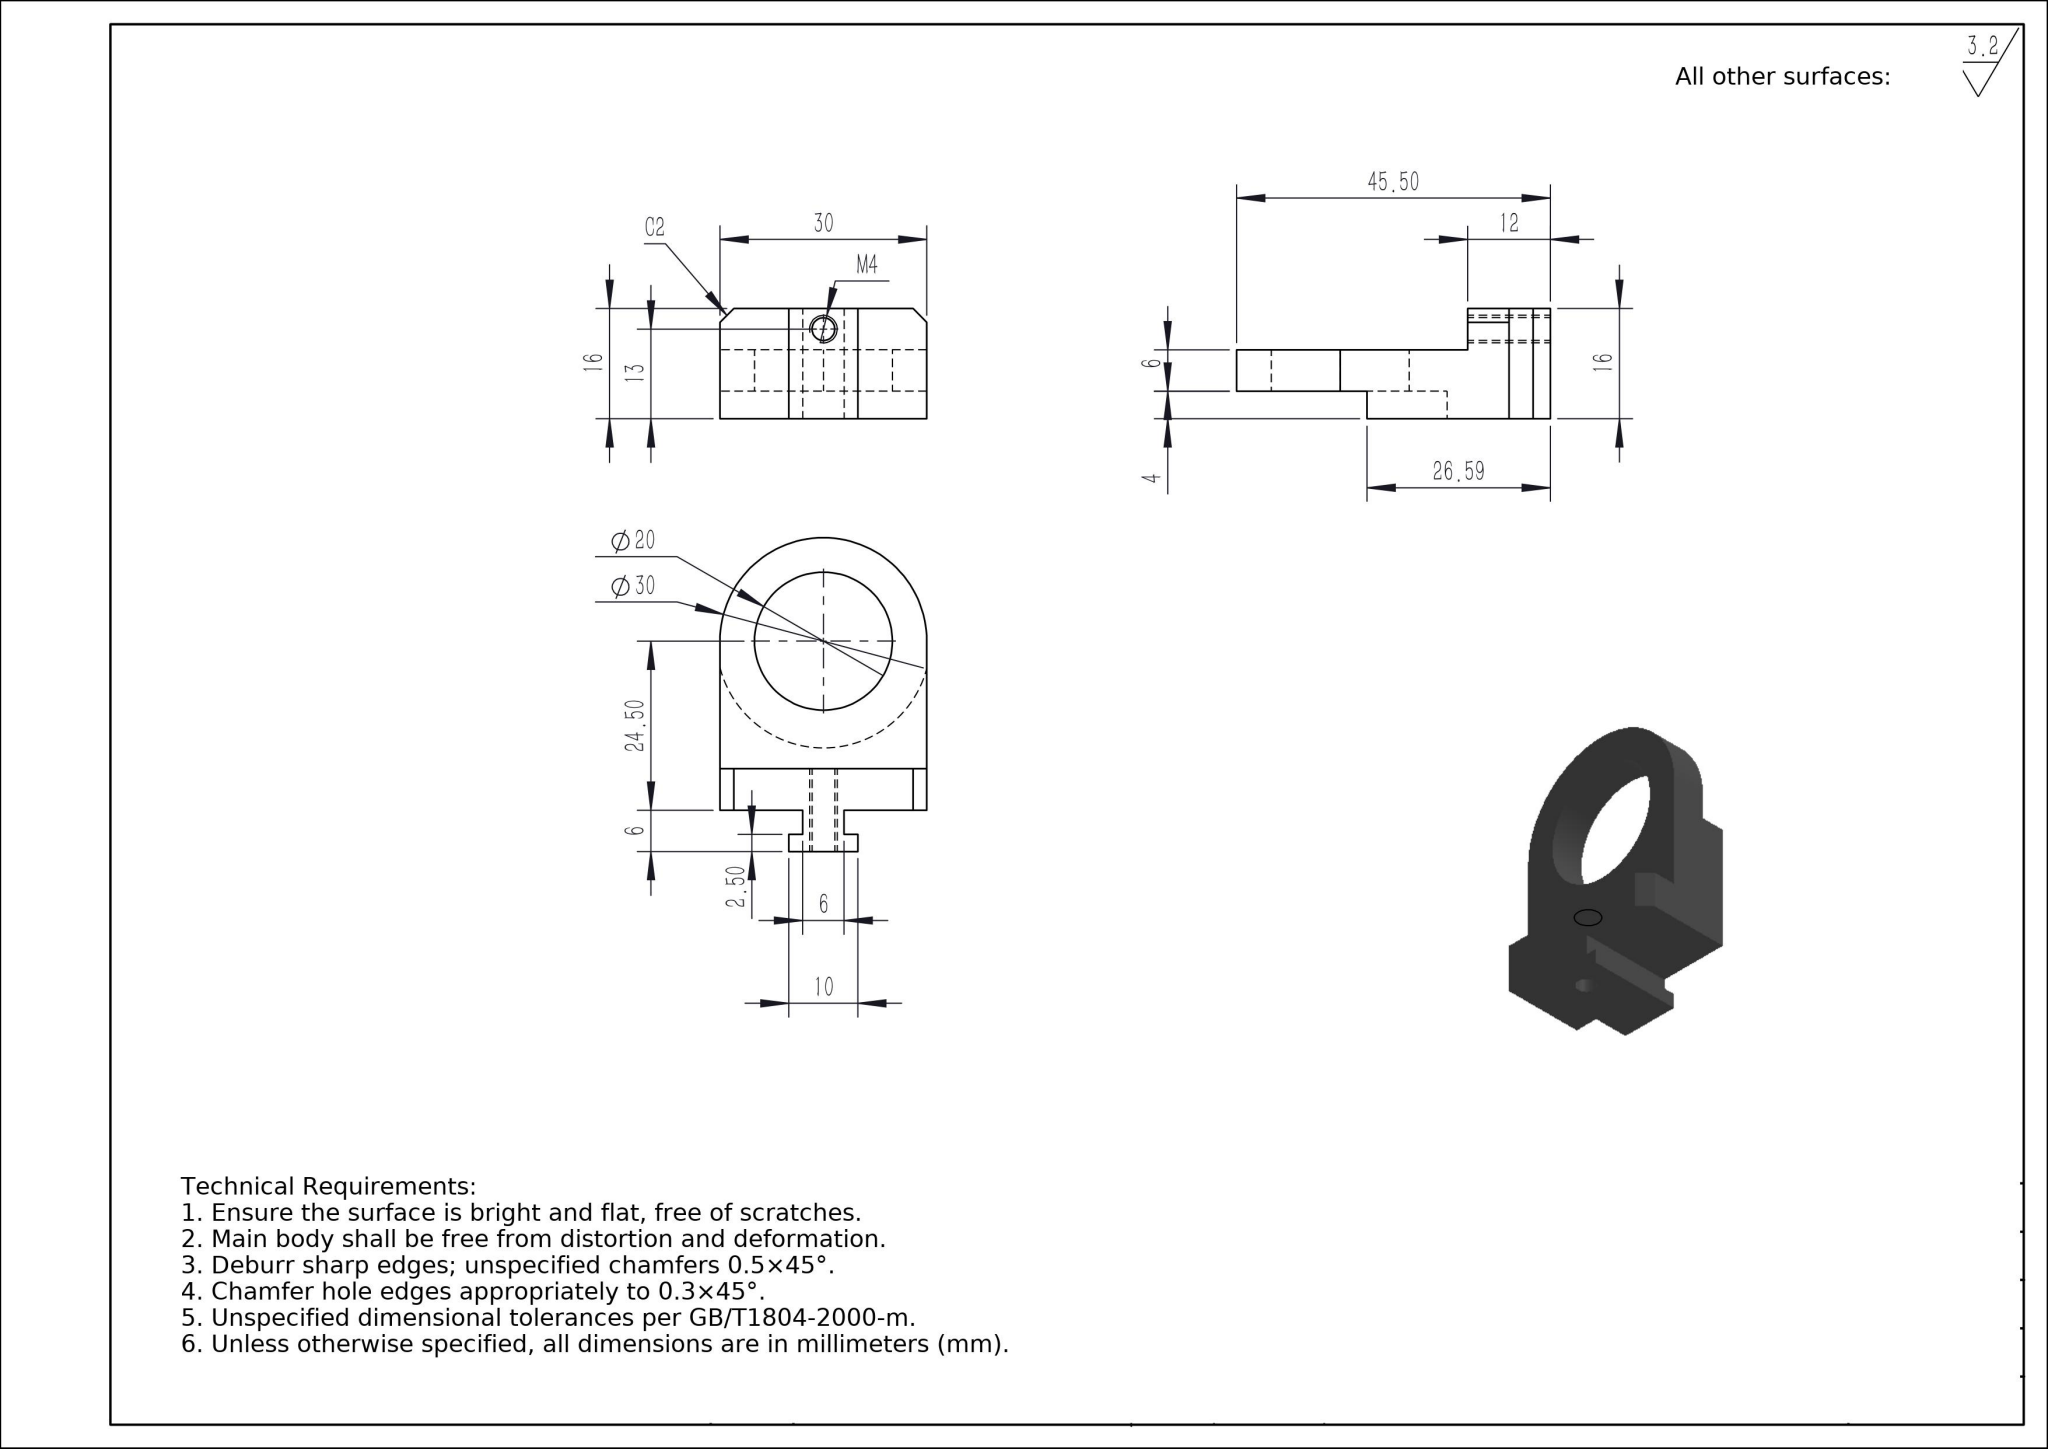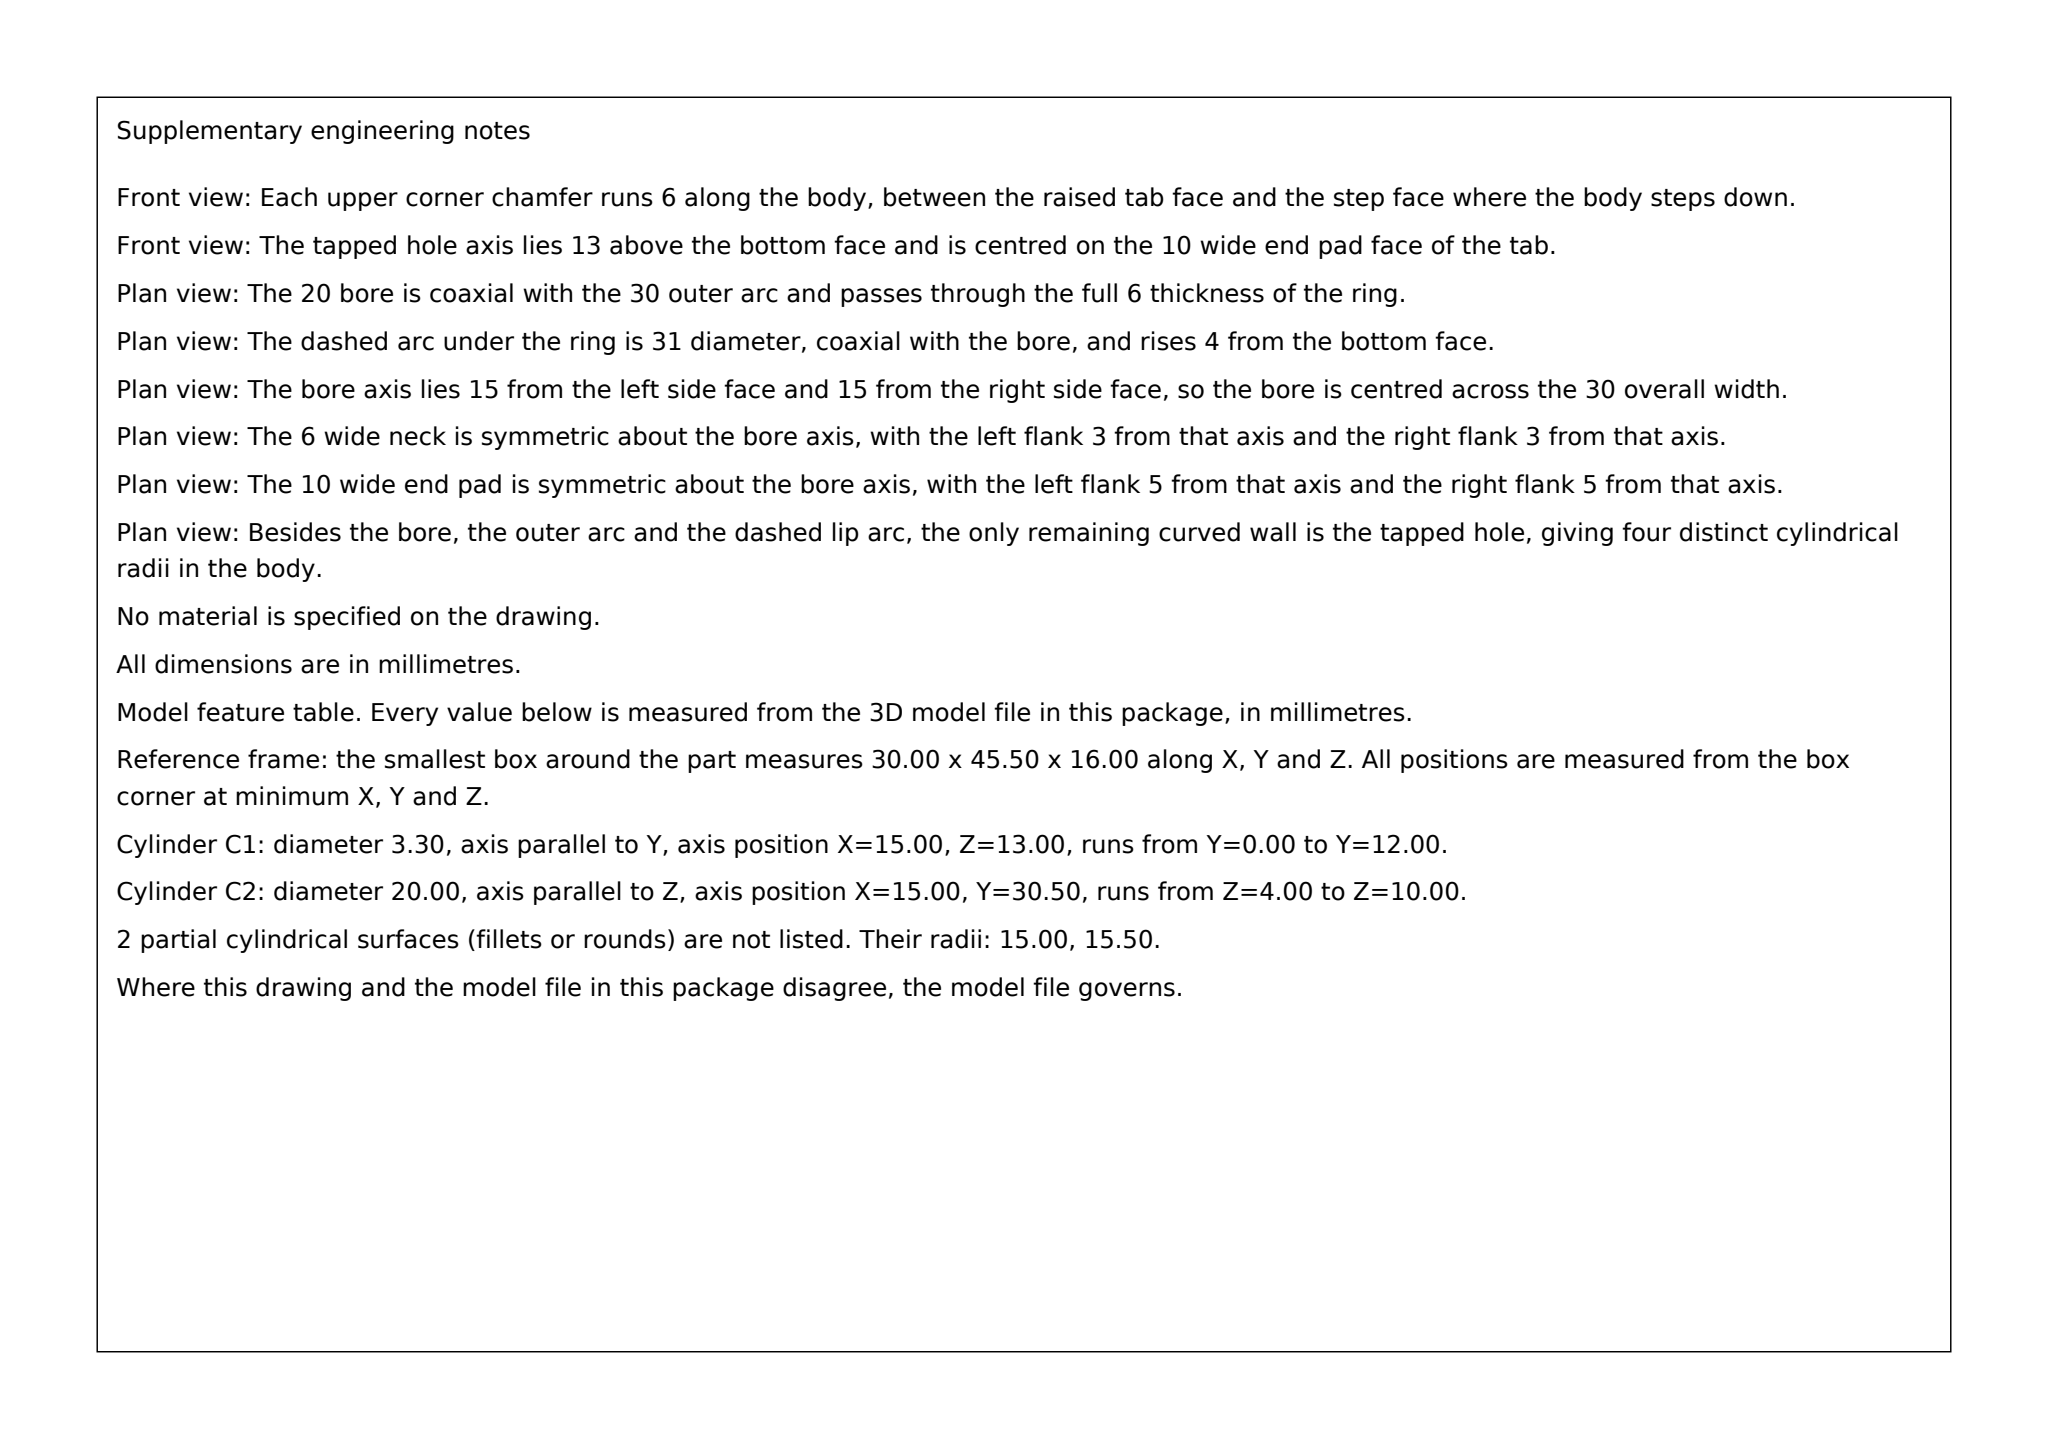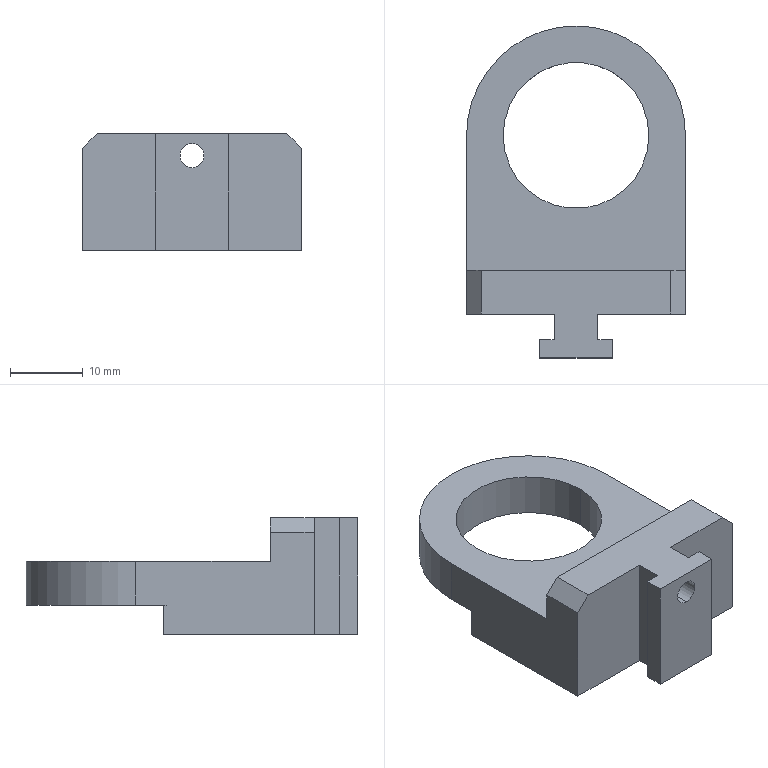Part | SolidWorks | mm | 1 solid | 25 faces | box 30 x 45.5 x 16 mm | volume 7776 mm3 | plane 18 | cylinder 7 | commonest cylinder face diameters 3.3 x2 20 x2 30 x2 31 x1
Drawing notes:
M4 TAPPED HOLE: 15 FROM EACH END OF 30 WIDTH (ON CL), 13 UP | from the solid: cylinder dia 3.3 axis y at x=15.0, z=13.0; bbox x=30.0 so x=15 is mid-width
R15.50 CONCAVE ARC COAXIAL W/ Ø30 BOSS, 4 DEEP FROM BOTTOM FACE | from the solid: concave arc dia 31.0 (R15.50), axis z at (15.0,30.5), from z=0.0 to z=4.0, 151 deg, same center as Ø30 convex arc and Ø20 bore
STEP:
#1=CARTESIAN_POINT('',(0.,-25.75,11.35));
#2=VERTEX_POINT('',#1);
#3=CARTESIAN_POINT('',(0.,-25.75,14.65));
#4=VERTEX_POINT('',#3);
#5=CARTESIAN_POINT('',(0.,-25.75,13.));
#6=DIRECTION('',(0.,1.,0.));
#7=DIRECTION('',(0.,0.,1.));
#8=AXIS2_PLACEMENT_3D('',#5,#6,#7);
#9=CIRCLE('',#8,1.65);
#10=EDGE_CURVE('',#2,#4,#9,.T.);
#11=ORIENTED_EDGE('',*,*,#10,.F.);
#12=CARTESIAN_POINT('',(0.,-13.75,11.35));
#13=VERTEX_POINT('',#12);
#14=CARTESIAN_POINT('',(0.,-13.75,11.35));
#15=DIRECTION('',(0.,1.,0.));
#16=VECTOR('',#15,1000.);
#17=LINE('',#14,#16);
#18=EDGE_CURVE('',#2,#13,#17,.T.);
#19=ORIENTED_EDGE('',*,*,#18,.T.);
#20=CARTESIAN_POINT('',(0.,-13.75,14.65));
#21=VERTEX_POINT('',#20);
#22=CARTESIAN_POINT('',(0.,-13.75,13.));
#23=DIRECTION('',(0.,1.,0.));
#24=DIRECTION('',(0.,0.,1.));
#25=AXIS2_PLACEMENT_3D('',#22,#23,#24);
#26=CIRCLE('',#25,1.65);
#27=EDGE_CURVE('',#13,#21,#26,.T.);
#28=ORIENTED_EDGE('',*,*,#27,.T.);
#29=CARTESIAN_POINT('',(0.,-13.75,14.65));
#30=DIRECTION('',(0.,1.,0.));
#31=VECTOR('',#30,1000.);
#32=LINE('',#29,#31);
#33=EDGE_CURVE('',#4,#21,#32,.T.);
#34=ORIENTED_EDGE('',*,*,#33,.F.);
#35=EDGE_LOOP('',(#11,#19,#28,#34));
#36=FACE_OUTER_BOUND('',#35,.T.);
#37=CARTESIAN_POINT('',(0.,-13.75,13.));
#38=DIRECTION('',(0.,1.,0.));
#39=DIRECTION('',(0.,0.,1.));
#40=AXIS2_PLACEMENT_3D('',#37,#38,#39);
#41=CYLINDRICAL_SURFACE('',#40,1.65);
#42=ADVANCED_FACE('',(#36),#41,.F.);
#43=CARTESIAN_POINT('',(-10.,4.75,4.));
#44=VERTEX_POINT('',#43);
#45=CARTESIAN_POINT('',(10.,4.75,4.));
#46=VERTEX_POINT('',#45);
#47=CARTESIAN_POINT('',(0.,4.75,4.));
#48=DIRECTION('',(0.,0.,1.));
#49=DIRECTION('',(-1.,0.,0.));
#50=AXIS2_PLACEMENT_3D('',#47,#48,#49);
#51=CIRCLE('',#50,10.);
#52=EDGE_CURVE('',#44,#46,#51,.T.);
#53=ORIENTED_EDGE('',*,*,#52,.F.);
#54=CARTESIAN_POINT('',(-10.,4.75,10.));
#55=VERTEX_POINT('',#54);
#56=CARTESIAN_POINT('',(-10.,4.75,-5.));
#57=DIRECTION('',(0.,0.,1.));
#58=VECTOR('',#57,1000.);
#59=LINE('',#56,#58);
#60=EDGE_CURVE('',#44,#55,#59,.T.);
#61=ORIENTED_EDGE('',*,*,#60,.T.);
#62=CARTESIAN_POINT('',(10.,4.75,10.));
#63=VERTEX_POINT('',#62);
#64=CARTESIAN_POINT('',(0.,4.75,10.));
#65=DIRECTION('',(0.,0.,1.));
#66=DIRECTION('',(1.,0.,0.));
#67=AXIS2_PLACEMENT_3D('',#64,#65,#66);
#68=CIRCLE('',#67,10.);
#69=EDGE_CURVE('',#55,#63,#68,.T.);
#70=ORIENTED_EDGE('',*,*,#69,.T.);
#71=CARTESIAN_POINT('',(10.,4.75,-5.));
#72=DIRECTION('',(0.,0.,1.));
#73=VECTOR('',#72,1000.);
#74=LINE('',#71,#73);
#75=EDGE_CURVE('',#46,#63,#74,.T.);
#76=ORIENTED_EDGE('',*,*,#75,.F.);
#77=EDGE_LOOP('',(#53,#61,#70,#76));
#78=FACE_OUTER_BOUND('',#77,.T.);
#79=CARTESIAN_POINT('',(0.,4.75,-5.));
#80=DIRECTION('',(0.,0.,1.));
#81=DIRECTION('',(1.,0.,0.));
#82=AXIS2_PLACEMENT_3D('',#79,#80,#81);
#83=CYLINDRICAL_SURFACE('',#82,10.);
#84=ADVANCED_FACE('',(#78),#83,.F.);
#85=CARTESIAN_POINT('',(-3.,-19.75,16.));
#86=VERTEX_POINT('',#85);
#87=CARTESIAN_POINT('',(-3.,-19.75,0.));
#88=VERTEX_POINT('',#87);
#89=CARTESIAN_POINT('',(-3.,-19.75,-0.));
#90=DIRECTION('',(0.,0.,-1.));
#91=VECTOR('',#90,1000.);
#92=LINE('',#89,#91);
#93=EDGE_CURVE('',#86,#88,#92,.T.);
#94=ORIENTED_EDGE('',*,*,#93,.F.);
#95=CARTESIAN_POINT('',(-13.,-19.75,16.));
#96=VERTEX_POINT('',#95);
#97=CARTESIAN_POINT('',(-15.,-19.75,16.));
#98=DIRECTION('',(1.,0.,0.));
#99=VECTOR('',#98,1000.);
#100=LINE('',#97,#99);
#101=EDGE_CURVE('',#96,#86,#100,.T.);
#102=ORIENTED_EDGE('',*,*,#101,.F.);
#103=CARTESIAN_POINT('',(-15.,-19.75,14.));
#104=VERTEX_POINT('',#103);
#105=CARTESIAN_POINT('',(-13.,-19.75,16.));
#106=DIRECTION('',(-0.7071,-0.,-0.7071));
#107=VECTOR('',#106,1000.);
#108=LINE('',#105,#107);
#109=EDGE_CURVE('',#96,#104,#108,.T.);
#110=ORIENTED_EDGE('',*,*,#109,.T.);
#111=CARTESIAN_POINT('',(-15.,-19.75,0.));
#112=VERTEX_POINT('',#111);
#113=CARTESIAN_POINT('',(-15.,-19.75,10.));
#114=DIRECTION('',(0.,0.,-1.));
#115=VECTOR('',#114,1000.);
#116=LINE('',#113,#115);
#117=EDGE_CURVE('',#104,#112,#116,.T.);
#118=ORIENTED_EDGE('',*,*,#117,.T.);
#119=CARTESIAN_POINT('',(15.,-19.75,0.));
#120=DIRECTION('',(1.,0.,0.));
#121=VECTOR('',#120,1000.);
#122=LINE('',#119,#121);
#123=EDGE_CURVE('',#112,#88,#122,.T.);
#124=ORIENTED_EDGE('',*,*,#123,.T.);
#125=EDGE_LOOP('',(#94,#102,#110,#118,#124));
#126=FACE_OUTER_BOUND('',#125,.T.);
#127=CARTESIAN_POINT('',(15.,-19.75,10.));
#128=DIRECTION('',(-0.,1.,0.));
#129=DIRECTION('',(-1.,-0.,0.));
#130=AXIS2_PLACEMENT_3D('',#127,#128,#129);
#131=PLANE('',#130);
#132=ADVANCED_FACE('',(#126),#131,.F.);
#133=CARTESIAN_POINT('',(3.,-19.75,0.));
#134=VERTEX_POINT('',#133);
#135=CARTESIAN_POINT('',(3.,-19.75,16.));
#136=VERTEX_POINT('',#135);
#137=CARTESIAN_POINT('',(3.,-19.75,-0.));
#138=DIRECTION('',(0.,0.,1.));
#139=VECTOR('',#138,1000.);
#140=LINE('',#137,#139);
#141=EDGE_CURVE('',#134,#136,#140,.T.);
#142=ORIENTED_EDGE('',*,*,#141,.F.);
#143=CARTESIAN_POINT('',(15.,-19.75,0.));
#144=VERTEX_POINT('',#143);
#145=CARTESIAN_POINT('',(15.,-19.75,0.));
#146=DIRECTION('',(1.,0.,0.));
#147=VECTOR('',#146,1000.);
#148=LINE('',#145,#147);
#149=EDGE_CURVE('',#134,#144,#148,.T.);
#150=ORIENTED_EDGE('',*,*,#149,.T.);
#151=CARTESIAN_POINT('',(15.,-19.75,14.));
#152=VERTEX_POINT('',#151);
#153=CARTESIAN_POINT('',(15.,-19.75,10.));
#154=DIRECTION('',(0.,0.,-1.));
#155=VECTOR('',#154,1000.);
#156=LINE('',#153,#155);
#157=EDGE_CURVE('',#152,#144,#156,.T.);
#158=ORIENTED_EDGE('',*,*,#157,.F.);
#159=CARTESIAN_POINT('',(13.,-19.75,16.));
#160=VERTEX_POINT('',#159);
#161=CARTESIAN_POINT('',(13.,-19.75,16.));
#162=DIRECTION('',(-0.7071,-0.,0.7071));
#163=VECTOR('',#162,1000.);
#164=LINE('',#161,#163);
#165=EDGE_CURVE('',#152,#160,#164,.T.);
#166=ORIENTED_EDGE('',*,*,#165,.T.);
#167=CARTESIAN_POINT('',(-15.,-19.75,16.));
#168=DIRECTION('',(1.,0.,0.));
#169=VECTOR('',#168,1000.);
#170=LINE('',#167,#169);
#171=EDGE_CURVE('',#136,#160,#170,.T.);
#172=ORIENTED_EDGE('',*,*,#171,.F.);
#173=EDGE_LOOP('',(#142,#150,#158,#166,#172));
#174=FACE_OUTER_BOUND('',#173,.T.);
#175=CARTESIAN_POINT('',(15.,-19.75,10.));
#176=DIRECTION('',(-0.,1.,0.));
#177=DIRECTION('',(-1.,-0.,0.));
#178=AXIS2_PLACEMENT_3D('',#175,#176,#177);
#179=PLANE('',#178);
#180=ADVANCED_FACE('',(#174),#179,.F.);
#181=CARTESIAN_POINT('',(-0.,19.75,4.));
#182=VERTEX_POINT('',#181);
#183=CARTESIAN_POINT('',(-0.,19.75,10.));
#184=VERTEX_POINT('',#183);
#185=CARTESIAN_POINT('',(-0.,19.75,10.));
#186=DIRECTION('',(0.,0.,1.));
#187=VECTOR('',#186,1000.);
#188=LINE('',#185,#187);
#189=EDGE_CURVE('',#182,#184,#188,.T.);
#190=ORIENTED_EDGE('',*,*,#189,.F.);
#191=CARTESIAN_POINT('',(-15.,4.75,4.));
#192=VERTEX_POINT('',#191);
#193=CARTESIAN_POINT('',(0.,4.75,4.));
#194=DIRECTION('',(0.,0.,1.));
#195=DIRECTION('',(-1.,-0.,0.));
#196=AXIS2_PLACEMENT_3D('',#193,#194,#195);
#197=CIRCLE('',#196,15.);
#198=EDGE_CURVE('',#182,#192,#197,.T.);
#199=ORIENTED_EDGE('',*,*,#198,.T.);
#200=CARTESIAN_POINT('',(-15.,4.75,10.));
#201=VERTEX_POINT('',#200);
#202=CARTESIAN_POINT('',(-15.,4.75,10.));
#203=DIRECTION('',(0.,0.,-1.));
#204=VECTOR('',#203,1000.);
#205=LINE('',#202,#204);
#206=EDGE_CURVE('',#201,#192,#205,.T.);
#207=ORIENTED_EDGE('',*,*,#206,.F.);
#208=CARTESIAN_POINT('',(0.,4.75,10.));
#209=DIRECTION('',(0.,0.,1.));
#210=DIRECTION('',(1.,0.,0.));
#211=AXIS2_PLACEMENT_3D('',#208,#209,#210);
#212=CIRCLE('',#211,15.);
#213=EDGE_CURVE('',#184,#201,#212,.T.);
#214=ORIENTED_EDGE('',*,*,#213,.F.);
#215=EDGE_LOOP('',(#190,#199,#207,#214));
#216=FACE_OUTER_BOUND('',#215,.T.);
#217=CARTESIAN_POINT('',(0.,4.75,10.));
#218=DIRECTION('',(0.,0.,-1.));
#219=DIRECTION('',(-1.,0.,0.));
#220=AXIS2_PLACEMENT_3D('',#217,#218,#219);
#221=CYLINDRICAL_SURFACE('',#220,15.);
#222=ADVANCED_FACE('',(#216),#221,.T.);
#223=CARTESIAN_POINT('',(15.,4.75,4.));
#224=VERTEX_POINT('',#223);
#225=CARTESIAN_POINT('',(15.,4.75,10.));
#226=VERTEX_POINT('',#225);
#227=CARTESIAN_POINT('',(15.,4.75,10.));
#228=DIRECTION('',(0.,0.,1.));
#229=VECTOR('',#228,1000.);
#230=LINE('',#227,#229);
#231=EDGE_CURVE('',#224,#226,#230,.T.);
#232=ORIENTED_EDGE('',*,*,#231,.F.);
#233=CARTESIAN_POINT('',(0.,4.75,4.));
#234=DIRECTION('',(0.,0.,1.));
#235=DIRECTION('',(-1.,0.,0.));
#236=AXIS2_PLACEMENT_3D('',#233,#234,#235);
#237=CIRCLE('',#236,15.);
#238=EDGE_CURVE('',#224,#182,#237,.T.);
#239=ORIENTED_EDGE('',*,*,#238,.T.);
#240=ORIENTED_EDGE('',*,*,#189,.T.);
#241=CARTESIAN_POINT('',(0.,4.75,10.));
#242=DIRECTION('',(0.,0.,1.));
#243=DIRECTION('',(1.,0.,0.));
#244=AXIS2_PLACEMENT_3D('',#241,#242,#243);
#245=CIRCLE('',#244,15.);
#246=EDGE_CURVE('',#226,#184,#245,.T.);
#247=ORIENTED_EDGE('',*,*,#246,.F.);
#248=EDGE_LOOP('',(#232,#239,#240,#247));
#249=FACE_OUTER_BOUND('',#248,.T.);
#250=CARTESIAN_POINT('',(0.,4.75,10.));
#251=DIRECTION('',(0.,0.,-1.));
#252=DIRECTION('',(-1.,0.,0.));
#253=AXIS2_PLACEMENT_3D('',#250,#251,#252);
#254=CYLINDRICAL_SURFACE('',#253,15.);
#255=ADVANCED_FACE('',(#249),#254,.T.);
#256=ORIENTED_EDGE('',*,*,#60,.F.);
#257=CARTESIAN_POINT('',(0.,4.75,4.));
#258=DIRECTION('',(0.,0.,1.));
#259=DIRECTION('',(-1.,0.,0.));
#260=AXIS2_PLACEMENT_3D('',#257,#258,#259);
#261=CIRCLE('',#260,10.);
#262=EDGE_CURVE('',#46,#44,#261,.T.);
#263=ORIENTED_EDGE('',*,*,#262,.F.);
#264=ORIENTED_EDGE('',*,*,#75,.T.);
#265=CARTESIAN_POINT('',(0.,4.75,10.));
#266=DIRECTION('',(0.,0.,1.));
#267=DIRECTION('',(1.,0.,0.));
#268=AXIS2_PLACEMENT_3D('',#265,#266,#267);
#269=CIRCLE('',#268,10.);
#270=EDGE_CURVE('',#63,#55,#269,.T.);
#271=ORIENTED_EDGE('',*,*,#270,.T.);
#272=EDGE_LOOP('',(#256,#263,#264,#271));
#273=FACE_OUTER_BOUND('',#272,.T.);
#274=CARTESIAN_POINT('',(0.,4.75,-5.));
#275=DIRECTION('',(0.,0.,1.));
#276=DIRECTION('',(1.,0.,0.));
#277=AXIS2_PLACEMENT_3D('',#274,#275,#276);
#278=CYLINDRICAL_SURFACE('',#277,10.);
#279=ADVANCED_FACE('',(#273),#278,.F.);
#280=ORIENTED_EDGE('',*,*,#117,.F.);
#281=CARTESIAN_POINT('',(-15.,-13.75,14.));
#282=VERTEX_POINT('',#281);
#283=CARTESIAN_POINT('',(-15.,-19.75,14.));
#284=DIRECTION('',(0.,1.,0.));
#285=VECTOR('',#284,1000.);
#286=LINE('',#283,#285);
#287=EDGE_CURVE('',#104,#282,#286,.T.);
#288=ORIENTED_EDGE('',*,*,#287,.T.);
#289=CARTESIAN_POINT('',(-15.,-13.75,10.));
#290=VERTEX_POINT('',#289);
#291=CARTESIAN_POINT('',(-15.,-13.75,16.));
#292=DIRECTION('',(0.,0.,-1.));
#293=VECTOR('',#292,1000.);
#294=LINE('',#291,#293);
#295=EDGE_CURVE('',#282,#290,#294,.T.);
#296=ORIENTED_EDGE('',*,*,#295,.T.);
#297=CARTESIAN_POINT('',(-15.,-19.75,10.));
#298=DIRECTION('',(0.,-1.,0.));
#299=VECTOR('',#298,1000.);
#300=LINE('',#297,#299);
#301=EDGE_CURVE('',#201,#290,#300,.T.);
#302=ORIENTED_EDGE('',*,*,#301,.F.);
#303=ORIENTED_EDGE('',*,*,#206,.T.);
#304=CARTESIAN_POINT('',(-15.,0.8449,4.));
#305=VERTEX_POINT('',#304);
#306=CARTESIAN_POINT('',(-15.,-19.75,4.));
#307=DIRECTION('',(0.,1.,0.));
#308=VECTOR('',#307,1000.);
#309=LINE('',#306,#308);
#310=EDGE_CURVE('',#305,#192,#309,.T.);
#311=ORIENTED_EDGE('',*,*,#310,.F.);
#312=CARTESIAN_POINT('',(-15.,0.8449,0.));
#313=VERTEX_POINT('',#312);
#314=CARTESIAN_POINT('',(-15.,0.8449,4.));
#315=DIRECTION('',(0.,0.,-1.));
#316=VECTOR('',#315,1000.);
#317=LINE('',#314,#316);
#318=EDGE_CURVE('',#305,#313,#317,.T.);
#319=ORIENTED_EDGE('',*,*,#318,.T.);
#320=CARTESIAN_POINT('',(-15.,-19.75,0.));
#321=DIRECTION('',(0.,-1.,0.));
#322=VECTOR('',#321,1000.);
#323=LINE('',#320,#322);
#324=EDGE_CURVE('',#313,#112,#323,.T.);
#325=ORIENTED_EDGE('',*,*,#324,.T.);
#326=EDGE_LOOP('',(#280,#288,#296,#302,#303,#311,#319,#325));
#327=FACE_OUTER_BOUND('',#326,.T.);
#328=CARTESIAN_POINT('',(-15.,-19.75,10.));
#329=DIRECTION('',(1.,0.,0.));
#330=DIRECTION('',(0.,0.,-1.));
#331=AXIS2_PLACEMENT_3D('',#328,#329,#330);
#332=PLANE('',#331);
#333=ADVANCED_FACE('',(#327),#332,.F.);
#334=CARTESIAN_POINT('',(15.,-13.75,14.));
#335=VERTEX_POINT('',#334);
#336=CARTESIAN_POINT('',(15.,-13.75,10.));
#337=VERTEX_POINT('',#336);
#338=CARTESIAN_POINT('',(15.,-13.75,16.));
#339=DIRECTION('',(0.,0.,-1.));
#340=VECTOR('',#339,1000.);
#341=LINE('',#338,#340);
#342=EDGE_CURVE('',#335,#337,#341,.T.);
#343=ORIENTED_EDGE('',*,*,#342,.F.);
#344=CARTESIAN_POINT('',(15.,-19.75,14.));
#345=DIRECTION('',(0.,-1.,0.));
#346=VECTOR('',#345,1000.);
#347=LINE('',#344,#346);
#348=EDGE_CURVE('',#335,#152,#347,.T.);
#349=ORIENTED_EDGE('',*,*,#348,.T.);
#350=ORIENTED_EDGE('',*,*,#157,.T.);
#351=CARTESIAN_POINT('',(15.,0.8449,0.));
#352=VERTEX_POINT('',#351);
#353=CARTESIAN_POINT('',(15.,-19.75,0.));
#354=DIRECTION('',(0.,1.,0.));
#355=VECTOR('',#354,1000.);
#356=LINE('',#353,#355);
#357=EDGE_CURVE('',#144,#352,#356,.T.);
#358=ORIENTED_EDGE('',*,*,#357,.T.);
#359=CARTESIAN_POINT('',(15.,0.8449,4.));
#360=VERTEX_POINT('',#359);
#361=CARTESIAN_POINT('',(15.,0.8449,4.));
#362=DIRECTION('',(0.,0.,1.));
#363=VECTOR('',#362,1000.);
#364=LINE('',#361,#363);
#365=EDGE_CURVE('',#352,#360,#364,.T.);
#366=ORIENTED_EDGE('',*,*,#365,.T.);
#367=CARTESIAN_POINT('',(15.,-19.75,4.));
#368=DIRECTION('',(0.,-1.,0.));
#369=VECTOR('',#368,1000.);
#370=LINE('',#367,#369);
#371=EDGE_CURVE('',#224,#360,#370,.T.);
#372=ORIENTED_EDGE('',*,*,#371,.F.);
#373=ORIENTED_EDGE('',*,*,#231,.T.);
#374=CARTESIAN_POINT('',(15.,-19.75,10.));
#375=DIRECTION('',(0.,1.,0.));
#376=VECTOR('',#375,1000.);
#377=LINE('',#374,#376);
#378=EDGE_CURVE('',#337,#226,#377,.T.);
#379=ORIENTED_EDGE('',*,*,#378,.F.);
#380=EDGE_LOOP('',(#343,#349,#350,#358,#366,#372,#373,#379));
#381=FACE_OUTER_BOUND('',#380,.T.);
#382=CARTESIAN_POINT('',(15.,-19.75,10.));
#383=DIRECTION('',(-1.,0.,0.));
#384=DIRECTION('',(0.,0.,1.));
#385=AXIS2_PLACEMENT_3D('',#382,#383,#384);
#386=PLANE('',#385);
#387=ADVANCED_FACE('',(#381),#386,.F.);
#388=CARTESIAN_POINT('',(-15.,-13.75,10.));
#389=DIRECTION('',(-1.,0.,0.));
#390=VECTOR('',#389,1000.);
#391=LINE('',#388,#390);
#392=EDGE_CURVE('',#337,#290,#391,.T.);
#393=ORIENTED_EDGE('',*,*,#392,.F.);
#394=ORIENTED_EDGE('',*,*,#378,.T.);
#395=ORIENTED_EDGE('',*,*,#246,.T.);
#396=ORIENTED_EDGE('',*,*,#213,.T.);
#397=ORIENTED_EDGE('',*,*,#301,.T.);
#398=EDGE_LOOP('',(#393,#394,#395,#396,#397));
#399=FACE_OUTER_BOUND('',#398,.T.);
#400=ORIENTED_EDGE('',*,*,#270,.F.);
#401=ORIENTED_EDGE('',*,*,#69,.F.);
#402=EDGE_LOOP('',(#400,#401));
#403=FACE_BOUND('',#402,.T.);
#404=CARTESIAN_POINT('',(0.,0.,10.));
#405=DIRECTION('',(0.,0.,1.));
#406=DIRECTION('',(1.,0.,0.));
#407=AXIS2_PLACEMENT_3D('',#404,#405,#406);
#408=PLANE('',#407);
#409=ADVANCED_FACE('',(#399,#403),#408,.T.);
#410=ORIENTED_EDGE('',*,*,#324,.F.);
#411=CARTESIAN_POINT('',(0.,4.75,0.));
#412=DIRECTION('',(0.,0.,-1.));
#413=DIRECTION('',(-1.,0.,0.));
#414=AXIS2_PLACEMENT_3D('',#411,#412,#413);
#415=CIRCLE('',#414,15.5);
#416=EDGE_CURVE('',#352,#313,#415,.T.);
#417=ORIENTED_EDGE('',*,*,#416,.F.);
#418=ORIENTED_EDGE('',*,*,#357,.F.);
#419=ORIENTED_EDGE('',*,*,#149,.F.);
#420=CARTESIAN_POINT('',(3.,-23.25,-0.));
#421=VERTEX_POINT('',#420);
#422=CARTESIAN_POINT('',(3.,-23.25,-0.));
#423=DIRECTION('',(-0.,1.,0.));
#424=VECTOR('',#423,1000.);
#425=LINE('',#422,#424);
#426=EDGE_CURVE('',#421,#134,#425,.T.);
#427=ORIENTED_EDGE('',*,*,#426,.F.);
#428=CARTESIAN_POINT('',(5.,-23.25,-0.));
#429=VERTEX_POINT('',#428);
#430=CARTESIAN_POINT('',(5.,-23.25,-0.));
#431=DIRECTION('',(1.,0.,0.));
#432=VECTOR('',#431,1000.);
#433=LINE('',#430,#432);
#434=EDGE_CURVE('',#421,#429,#433,.T.);
#435=ORIENTED_EDGE('',*,*,#434,.T.);
#436=CARTESIAN_POINT('',(5.,-25.75,-0.));
#437=VERTEX_POINT('',#436);
#438=CARTESIAN_POINT('',(5.,-25.75,-0.));
#439=DIRECTION('',(0.,1.,0.));
#440=VECTOR('',#439,1000.);
#441=LINE('',#438,#440);
#442=EDGE_CURVE('',#437,#429,#441,.T.);
#443=ORIENTED_EDGE('',*,*,#442,.F.);
#444=CARTESIAN_POINT('',(-5.,-25.75,-0.));
#445=VERTEX_POINT('',#444);
#446=CARTESIAN_POINT('',(5.,-25.75,-0.));
#447=DIRECTION('',(1.,0.,0.));
#448=VECTOR('',#447,1000.);
#449=LINE('',#446,#448);
#450=EDGE_CURVE('',#445,#437,#449,.T.);
#451=ORIENTED_EDGE('',*,*,#450,.F.);
#452=CARTESIAN_POINT('',(-5.,-23.25,-0.));
#453=VERTEX_POINT('',#452);
#454=CARTESIAN_POINT('',(-5.,-25.75,-0.));
#455=DIRECTION('',(0.,1.,0.));
#456=VECTOR('',#455,1000.);
#457=LINE('',#454,#456);
#458=EDGE_CURVE('',#445,#453,#457,.T.);
#459=ORIENTED_EDGE('',*,*,#458,.T.);
#460=CARTESIAN_POINT('',(-3.,-23.25,-0.));
#461=VERTEX_POINT('',#460);
#462=CARTESIAN_POINT('',(5.,-23.25,-0.));
#463=DIRECTION('',(1.,0.,0.));
#464=VECTOR('',#463,1000.);
#465=LINE('',#462,#464);
#466=EDGE_CURVE('',#453,#461,#465,.T.);
#467=ORIENTED_EDGE('',*,*,#466,.T.);
#468=CARTESIAN_POINT('',(-3.,-23.25,-0.));
#469=DIRECTION('',(-0.,1.,0.));
#470=VECTOR('',#469,1000.);
#471=LINE('',#468,#470);
#472=EDGE_CURVE('',#461,#88,#471,.T.);
#473=ORIENTED_EDGE('',*,*,#472,.T.);
#474=ORIENTED_EDGE('',*,*,#123,.F.);
#475=EDGE_LOOP('',(#410,#417,#418,#419,#427,#435,#443,#451,#459,#467,#473,#474));
#476=FACE_OUTER_BOUND('',#475,.T.);
#477=CARTESIAN_POINT('',(0.,0.,0.));
#478=DIRECTION('',(0.,0.,1.));
#479=DIRECTION('',(1.,0.,0.));
#480=AXIS2_PLACEMENT_3D('',#477,#478,#479);
#481=PLANE('',#480);
#482=ADVANCED_FACE('',(#476),#481,.F.);
#483=CARTESIAN_POINT('',(0.,4.75,4.));
#484=DIRECTION('',(0.,0.,-1.));
#485=DIRECTION('',(-1.,0.,0.));
#486=AXIS2_PLACEMENT_3D('',#483,#484,#485);
#487=CIRCLE('',#486,15.5);
#488=EDGE_CURVE('',#360,#305,#487,.T.);
#489=ORIENTED_EDGE('',*,*,#488,.F.);
#490=ORIENTED_EDGE('',*,*,#365,.F.);
#491=ORIENTED_EDGE('',*,*,#416,.T.);
#492=ORIENTED_EDGE('',*,*,#318,.F.);
#493=EDGE_LOOP('',(#489,#490,#491,#492));
#494=FACE_OUTER_BOUND('',#493,.T.);
#495=CARTESIAN_POINT('',(0.,4.75,4.));
#496=DIRECTION('',(0.,0.,-1.));
#497=DIRECTION('',(-1.,0.,0.));
#498=AXIS2_PLACEMENT_3D('',#495,#496,#497);
#499=CYLINDRICAL_SURFACE('',#498,15.5);
#500=ADVANCED_FACE('',(#494),#499,.F.);
#501=ORIENTED_EDGE('',*,*,#262,.T.);
#502=ORIENTED_EDGE('',*,*,#52,.T.);
#503=EDGE_LOOP('',(#501,#502));
#504=FACE_BOUND('',#503,.T.);
#505=ORIENTED_EDGE('',*,*,#310,.T.);
#506=ORIENTED_EDGE('',*,*,#198,.F.);
#507=ORIENTED_EDGE('',*,*,#238,.F.);
#508=ORIENTED_EDGE('',*,*,#371,.T.);
#509=ORIENTED_EDGE('',*,*,#488,.T.);
#510=EDGE_LOOP('',(#505,#506,#507,#508,#509));
#511=FACE_OUTER_BOUND('',#510,.T.);
#512=CARTESIAN_POINT('',(0.,4.75,4.));
#513=DIRECTION('',(0.,0.,-1.));
#514=DIRECTION('',(-1.,0.,0.));
#515=AXIS2_PLACEMENT_3D('',#512,#513,#514);
#516=PLANE('',#515);
#517=ADVANCED_FACE('',(#504,#511),#516,.T.);
#518=CARTESIAN_POINT('',(0.,-13.75,13.));
#519=DIRECTION('',(0.,1.,0.));
#520=DIRECTION('',(0.,0.,1.));
#521=AXIS2_PLACEMENT_3D('',#518,#519,#520);
#522=CIRCLE('',#521,1.65);
#523=EDGE_CURVE('',#21,#13,#522,.T.);
#524=ORIENTED_EDGE('',*,*,#523,.F.);
#525=ORIENTED_EDGE('',*,*,#27,.F.);
#526=EDGE_LOOP('',(#524,#525));
#527=FACE_BOUND('',#526,.T.);
#528=ORIENTED_EDGE('',*,*,#295,.F.);
#529=CARTESIAN_POINT('',(-13.,-13.75,16.));
#530=VERTEX_POINT('',#529);
#531=CARTESIAN_POINT('',(-13.,-13.75,16.));
#532=DIRECTION('',(0.7071,0.,0.7071));
#533=VECTOR('',#532,1000.);
#534=LINE('',#531,#533);
#535=EDGE_CURVE('',#282,#530,#534,.T.);
#536=ORIENTED_EDGE('',*,*,#535,.T.);
#537=CARTESIAN_POINT('',(13.,-13.75,16.));
#538=VERTEX_POINT('',#537);
#539=CARTESIAN_POINT('',(-15.,-13.75,16.));
#540=DIRECTION('',(-1.,0.,0.));
#541=VECTOR('',#540,1000.);
#542=LINE('',#539,#541);
#543=EDGE_CURVE('',#538,#530,#542,.T.);
#544=ORIENTED_EDGE('',*,*,#543,.F.);
#545=CARTESIAN_POINT('',(13.,-13.75,16.));
#546=DIRECTION('',(0.7071,0.,-0.7071));
#547=VECTOR('',#546,1000.);
#548=LINE('',#545,#547);
#549=EDGE_CURVE('',#538,#335,#548,.T.);
#550=ORIENTED_EDGE('',*,*,#549,.T.);
#551=ORIENTED_EDGE('',*,*,#342,.T.);
#552=ORIENTED_EDGE('',*,*,#392,.T.);
#553=EDGE_LOOP('',(#528,#536,#544,#550,#551,#552));
#554=FACE_OUTER_BOUND('',#553,.T.);
#555=CARTESIAN_POINT('',(-15.,-13.75,16.));
#556=DIRECTION('',(0.,-1.,0.));
#557=DIRECTION('',(0.,0.,-1.));
#558=AXIS2_PLACEMENT_3D('',#555,#556,#557);
#559=PLANE('',#558);
#560=ADVANCED_FACE('',(#527,#554),#559,.F.);
#561=ORIENTED_EDGE('',*,*,#543,.T.);
#562=CARTESIAN_POINT('',(-13.,0.,16.));
#563=DIRECTION('',(0.,-1.,0.));
#564=VECTOR('',#563,1000.);
#565=LINE('',#562,#564);
#566=EDGE_CURVE('',#530,#96,#565,.T.);
#567=ORIENTED_EDGE('',*,*,#566,.T.);
#568=ORIENTED_EDGE('',*,*,#101,.T.);
#569=CARTESIAN_POINT('',(-3.,-23.25,16.));
#570=VERTEX_POINT('',#569);
#571=CARTESIAN_POINT('',(-3.,-23.25,16.));
#572=DIRECTION('',(-0.,1.,0.));
#573=VECTOR('',#572,1000.);
#574=LINE('',#571,#573);
#575=EDGE_CURVE('',#570,#86,#574,.T.);
#576=ORIENTED_EDGE('',*,*,#575,.F.);
#577=CARTESIAN_POINT('',(-5.,-23.25,16.));
#578=VERTEX_POINT('',#577);
#579=CARTESIAN_POINT('',(5.,-23.25,16.));
#580=DIRECTION('',(-1.,0.,0.));
#581=VECTOR('',#580,1000.);
#582=LINE('',#579,#581);
#583=EDGE_CURVE('',#570,#578,#582,.T.);
#584=ORIENTED_EDGE('',*,*,#583,.T.);
#585=CARTESIAN_POINT('',(-5.,-25.75,16.));
#586=VERTEX_POINT('',#585);
#587=CARTESIAN_POINT('',(-5.,-25.75,16.));
#588=DIRECTION('',(0.,1.,0.));
#589=VECTOR('',#588,1000.);
#590=LINE('',#587,#589);
#591=EDGE_CURVE('',#586,#578,#590,.T.);
#592=ORIENTED_EDGE('',*,*,#591,.F.);
#593=CARTESIAN_POINT('',(5.,-25.75,16.));
#594=VERTEX_POINT('',#593);
#595=CARTESIAN_POINT('',(5.,-25.75,16.));
#596=DIRECTION('',(-1.,0.,0.));
#597=VECTOR('',#596,1000.);
#598=LINE('',#595,#597);
#599=EDGE_CURVE('',#594,#586,#598,.T.);
#600=ORIENTED_EDGE('',*,*,#599,.F.);
#601=CARTESIAN_POINT('',(5.,-23.25,16.));
#602=VERTEX_POINT('',#601);
#603=CARTESIAN_POINT('',(5.,-25.75,16.));
#604=DIRECTION('',(0.,1.,0.));
#605=VECTOR('',#604,1000.);
#606=LINE('',#603,#605);
#607=EDGE_CURVE('',#594,#602,#606,.T.);
#608=ORIENTED_EDGE('',*,*,#607,.T.);
#609=CARTESIAN_POINT('',(3.,-23.25,16.));
#610=VERTEX_POINT('',#609);
#611=CARTESIAN_POINT('',(5.,-23.25,16.));
#612=DIRECTION('',(-1.,0.,0.));
#613=VECTOR('',#612,1000.);
#614=LINE('',#611,#613);
#615=EDGE_CURVE('',#602,#610,#614,.T.);
#616=ORIENTED_EDGE('',*,*,#615,.T.);
#617=CARTESIAN_POINT('',(3.,-23.25,16.));
#618=DIRECTION('',(-0.,1.,0.));
#619=VECTOR('',#618,1000.);
#620=LINE('',#617,#619);
#621=EDGE_CURVE('',#610,#136,#620,.T.);
#622=ORIENTED_EDGE('',*,*,#621,.T.);
#623=ORIENTED_EDGE('',*,*,#171,.T.);
#624=CARTESIAN_POINT('',(13.,0.,16.));
#625=DIRECTION('',(0.,1.,0.));
#626=VECTOR('',#625,1000.);
#627=LINE('',#624,#626);
#628=EDGE_CURVE('',#160,#538,#627,.T.);
#629=ORIENTED_EDGE('',*,*,#628,.T.);
#630=EDGE_LOOP('',(#561,#567,#568,#576,#584,#592,#600,#608,#616,#622,#623,#629));
#631=FACE_OUTER_BOUND('',#630,.T.);
#632=CARTESIAN_POINT('',(0.,0.,16.));
#633=DIRECTION('',(0.,0.,-1.));
#634=DIRECTION('',(-1.,0.,0.));
#635=AXIS2_PLACEMENT_3D('',#632,#633,#634);
#636=PLANE('',#635);
#637=ADVANCED_FACE('',(#631),#636,.F.);
#638=ORIENTED_EDGE('',*,*,#535,.F.);
#639=ORIENTED_EDGE('',*,*,#287,.F.);
#640=ORIENTED_EDGE('',*,*,#109,.F.);
#641=ORIENTED_EDGE('',*,*,#566,.F.);
#642=EDGE_LOOP('',(#638,#639,#640,#641));
#643=FACE_OUTER_BOUND('',#642,.T.);
#644=CARTESIAN_POINT('',(-13.,0.,16.));
#645=DIRECTION('',(0.7071,0.,-0.7071));
#646=DIRECTION('',(0.,-1.,0.));
#647=AXIS2_PLACEMENT_3D('',#644,#645,#646);
#648=PLANE('',#647);
#649=ADVANCED_FACE('',(#643),#648,.F.);
#650=ORIENTED_EDGE('',*,*,#165,.F.);
#651=ORIENTED_EDGE('',*,*,#348,.F.);
#652=ORIENTED_EDGE('',*,*,#549,.F.);
#653=ORIENTED_EDGE('',*,*,#628,.F.);
#654=EDGE_LOOP('',(#650,#651,#652,#653));
#655=FACE_OUTER_BOUND('',#654,.T.);
#656=CARTESIAN_POINT('',(13.,0.,16.));
#657=DIRECTION('',(-0.7071,0.,-0.7071));
#658=DIRECTION('',(0.,1.,0.));
#659=AXIS2_PLACEMENT_3D('',#656,#657,#658);
#660=PLANE('',#659);
#661=ADVANCED_FACE('',(#655),#660,.F.);
#662=ORIENTED_EDGE('',*,*,#93,.T.);
#663=ORIENTED_EDGE('',*,*,#472,.F.);
#664=CARTESIAN_POINT('',(-3.,-23.25,-0.));
#665=DIRECTION('',(0.,0.,-1.));
#666=VECTOR('',#665,1000.);
#667=LINE('',#664,#666);
#668=EDGE_CURVE('',#570,#461,#667,.T.);
#669=ORIENTED_EDGE('',*,*,#668,.F.);
#670=ORIENTED_EDGE('',*,*,#575,.T.);
#671=EDGE_LOOP('',(#662,#663,#669,#670));
#672=FACE_OUTER_BOUND('',#671,.T.);
#673=CARTESIAN_POINT('',(-3.,-23.25,-0.));
#674=DIRECTION('',(1.,0.,0.));
#675=DIRECTION('',(-0.,1.,0.));
#676=AXIS2_PLACEMENT_3D('',#673,#674,#675);
#677=PLANE('',#676);
#678=ADVANCED_FACE('',(#672),#677,.F.);
#679=ORIENTED_EDGE('',*,*,#141,.T.);
#680=ORIENTED_EDGE('',*,*,#621,.F.);
#681=CARTESIAN_POINT('',(3.,-23.25,-0.));
#682=DIRECTION('',(0.,0.,1.));
#683=VECTOR('',#682,1000.);
#684=LINE('',#681,#683);
#685=EDGE_CURVE('',#421,#610,#684,.T.);
#686=ORIENTED_EDGE('',*,*,#685,.F.);
#687=ORIENTED_EDGE('',*,*,#426,.T.);
#688=EDGE_LOOP('',(#679,#680,#686,#687));
#689=FACE_OUTER_BOUND('',#688,.T.);
#690=CARTESIAN_POINT('',(3.,-23.25,-0.));
#691=DIRECTION('',(-1.,-0.,0.));
#692=DIRECTION('',(0.,-1.,0.));
#693=AXIS2_PLACEMENT_3D('',#690,#691,#692);
#694=PLANE('',#693);
#695=ADVANCED_FACE('',(#689),#694,.F.);
#696=ORIENTED_EDGE('',*,*,#583,.F.);
#697=ORIENTED_EDGE('',*,*,#668,.T.);
#698=ORIENTED_EDGE('',*,*,#466,.F.);
#699=CARTESIAN_POINT('',(-5.,-23.25,-0.));
#700=DIRECTION('',(0.,0.,-1.));
#701=VECTOR('',#700,1000.);
#702=LINE('',#699,#701);
#703=EDGE_CURVE('',#578,#453,#702,.T.);
#704=ORIENTED_EDGE('',*,*,#703,.F.);
#705=EDGE_LOOP('',(#696,#697,#698,#704));
#706=FACE_OUTER_BOUND('',#705,.T.);
#707=CARTESIAN_POINT('',(0.,-23.25,0.));
#708=DIRECTION('',(0.,-1.,0.));
#709=DIRECTION('',(0.,0.,-1.));
#710=AXIS2_PLACEMENT_3D('',#707,#708,#709);
#711=PLANE('',#710);
#712=ADVANCED_FACE('',(#706),#711,.F.);
#713=ORIENTED_EDGE('',*,*,#434,.F.);
#714=ORIENTED_EDGE('',*,*,#685,.T.);
#715=ORIENTED_EDGE('',*,*,#615,.F.);
#716=CARTESIAN_POINT('',(5.,-23.25,-0.));
#717=DIRECTION('',(-0.,0.,1.));
#718=VECTOR('',#717,1000.);
#719=LINE('',#716,#718);
#720=EDGE_CURVE('',#429,#602,#719,.T.);
#721=ORIENTED_EDGE('',*,*,#720,.F.);
#722=EDGE_LOOP('',(#713,#714,#715,#721));
#723=FACE_OUTER_BOUND('',#722,.T.);
#724=CARTESIAN_POINT('',(0.,-23.25,0.));
#725=DIRECTION('',(0.,-1.,0.));
#726=DIRECTION('',(0.,0.,-1.));
#727=AXIS2_PLACEMENT_3D('',#724,#725,#726);
#728=PLANE('',#727);
#729=ADVANCED_FACE('',(#723),#728,.F.);
#730=ORIENTED_EDGE('',*,*,#703,.T.);
#731=ORIENTED_EDGE('',*,*,#458,.F.);
#732=CARTESIAN_POINT('',(-5.,-25.75,-0.));
#733=DIRECTION('',(0.,0.,-1.));
#734=VECTOR('',#733,1000.);
#735=LINE('',#732,#734);
#736=EDGE_CURVE('',#586,#445,#735,.T.);
#737=ORIENTED_EDGE('',*,*,#736,.F.);
#738=ORIENTED_EDGE('',*,*,#591,.T.);
#739=EDGE_LOOP('',(#730,#731,#737,#738));
#740=FACE_OUTER_BOUND('',#739,.T.);
#741=CARTESIAN_POINT('',(-5.,-25.75,-0.));
#742=DIRECTION('',(1.,0.,0.));
#743=DIRECTION('',(0.,0.,-1.));
#744=AXIS2_PLACEMENT_3D('',#741,#742,#743);
#745=PLANE('',#744);
#746=ADVANCED_FACE('',(#740),#745,.F.);
#747=ORIENTED_EDGE('',*,*,#720,.T.);
#748=ORIENTED_EDGE('',*,*,#607,.F.);
#749=CARTESIAN_POINT('',(5.,-25.75,-0.));
#750=DIRECTION('',(-0.,0.,1.));
#751=VECTOR('',#750,1000.);
#752=LINE('',#749,#751);
#753=EDGE_CURVE('',#437,#594,#752,.T.);
#754=ORIENTED_EDGE('',*,*,#753,.F.);
#755=ORIENTED_EDGE('',*,*,#442,.T.);
#756=EDGE_LOOP('',(#747,#748,#754,#755));
#757=FACE_OUTER_BOUND('',#756,.T.);
#758=CARTESIAN_POINT('',(5.,-25.75,-0.));
#759=DIRECTION('',(-1.,0.,-0.));
#760=DIRECTION('',(-0.,0.,1.));
#761=AXIS2_PLACEMENT_3D('',#758,#759,#760);
#762=PLANE('',#761);
#763=ADVANCED_FACE('',(#757),#762,.F.);
#764=CARTESIAN_POINT('',(0.,-25.75,13.));
#765=DIRECTION('',(0.,1.,0.));
#766=DIRECTION('',(0.,0.,1.));
#767=AXIS2_PLACEMENT_3D('',#764,#765,#766);
#768=CIRCLE('',#767,1.65);
#769=EDGE_CURVE('',#4,#2,#768,.T.);
#770=ORIENTED_EDGE('',*,*,#769,.T.);
#771=ORIENTED_EDGE('',*,*,#10,.T.);
#772=EDGE_LOOP('',(#770,#771));
#773=FACE_BOUND('',#772,.T.);
#774=ORIENTED_EDGE('',*,*,#736,.T.);
#775=ORIENTED_EDGE('',*,*,#450,.T.);
#776=ORIENTED_EDGE('',*,*,#753,.T.);
#777=ORIENTED_EDGE('',*,*,#599,.T.);
#778=EDGE_LOOP('',(#774,#775,#776,#777));
#779=FACE_OUTER_BOUND('',#778,.T.);
#780=CARTESIAN_POINT('',(0.,-25.75,0.));
#781=DIRECTION('',(0.,-1.,0.));
#782=DIRECTION('',(0.,0.,-1.));
#783=AXIS2_PLACEMENT_3D('',#780,#781,#782);
#784=PLANE('',#783);
#785=ADVANCED_FACE('',(#773,#779),#784,.T.);
#786=ORIENTED_EDGE('',*,*,#18,.F.);
#787=ORIENTED_EDGE('',*,*,#769,.F.);
#788=ORIENTED_EDGE('',*,*,#33,.T.);
#789=ORIENTED_EDGE('',*,*,#523,.T.);
#790=EDGE_LOOP('',(#786,#787,#788,#789));
#791=FACE_OUTER_BOUND('',#790,.T.);
#792=CARTESIAN_POINT('',(0.,-13.75,13.));
#793=DIRECTION('',(0.,1.,0.));
#794=DIRECTION('',(0.,0.,1.));
#795=AXIS2_PLACEMENT_3D('',#792,#793,#794);
#796=CYLINDRICAL_SURFACE('',#795,1.65);
#797=ADVANCED_FACE('',(#791),#796,.F.);
#798=CLOSED_SHELL('',(#42,#84,#132,#180,#222,#255,#279,#333,#387,#409,#482,#500,#517,#560,#637,#649,#661,#678,#695,#712,#729,#746,#763,#785,#797));
#799=MANIFOLD_SOLID_BREP('',#798);
#800=CARTESIAN_POINT('',(0.,0.,0.));
#801=DIRECTION('',(0.,0.,1.));
#802=DIRECTION('',(1.,0.,0.));
#803=AXIS2_PLACEMENT_3D('',#800,#801,#802);
#804=(LENGTH_UNIT()NAMED_UNIT(*)SI_UNIT(.MILLI.,.METRE.));
#805=UNCERTAINTY_MEASURE_WITH_UNIT(LENGTH_MEASURE(0.00001),#804,'','');
#806=(NAMED_UNIT(*)PLANE_ANGLE_UNIT()SI_UNIT($,.RADIAN.));
#807=(NAMED_UNIT(*)SI_UNIT($,.STERADIAN.)SOLID_ANGLE_UNIT());
#808=(GEOMETRIC_REPRESENTATION_CONTEXT(3)GLOBAL_UNCERTAINTY_ASSIGNED_CONTEXT((#805))GLOBAL_UNIT_ASSIGNED_CONTEXT((#804,#806,#807))REPRESENTATION_CONTEXT('',''));
#809=ADVANCED_BREP_SHAPE_REPRESENTATION('',(#799,#803),#808);